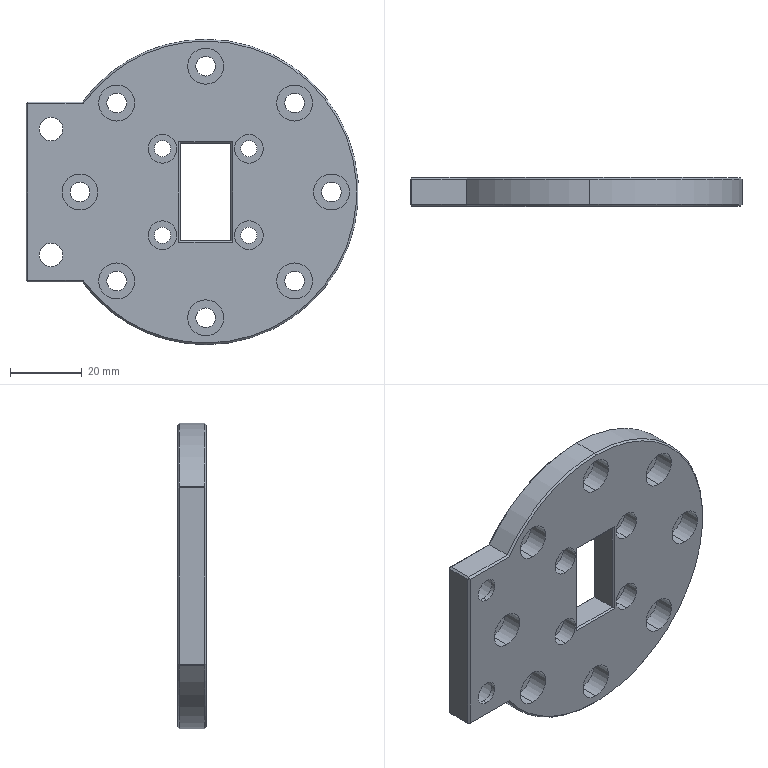Component | SolidWorks | BearingHousingAssembly-1_AirGripperFixingPlate1-1 | 1 solid | 108 faces | box 92.5 x 8 x 85 mm | volume 39781 mm3 | cylinder 59 | plane 43 | cone 6 | commonest cylinder face diameters 10 x16 5.5 x16 8 x8 4.5 x8 11 x4 6.6 x4 85 x3 | material Plain Carbon Steel
build123d program:
from build123d import *

# Parameters (mm, degrees)
SKETCH1_R                                          = 42.5
SKETCH1_W                                          = 27
SKETCH1_H                                          = 14
BOSS_EXTRUDE1_DEPTH                                = 8
HOLE_SIZE_ACCORDING_TO_TYPE_OF_HEXAGON_D           = 5.5
HOLE_SIZE_ACCORDING_TO_TYPE_OF_HEXAGON_CBORE_D     = 10
HOLE_SIZE_ACCORDING_TO_TYPE_OF_HEXAGON_CBORE_DEPTH = 5.7
CIRPATTERN1_COUNT                                  = 8
BOSS_EXTRUDE2_START                                = -8
BOSS_EXTRUDE2_DEPTH                                = 8
HOLE_SIZE_ACCORDING_TO_TYPE_OF_HEX_2_D             = 6.6
HOLE_SIZE_ACCORDING_TO_TYPE_OF_HEX_2_CBORE_D       = 11
HOLE_SIZE_ACCORDING_TO_TYPE_OF_HEX_2_CBORE_DEPTH   = 6.8
CHAMFER1_SIZE                                      = 0.5
CIRPATTERN2_COUNT                                  = 4


with BuildPart() as part:
    # Sketch1 → Boss-Extrude1 (new body)
    with BuildSketch(Plane.XY):
        Circle(SKETCH1_R)
        Rectangle(SKETCH1_W, SKETCH1_H, mode=Mode.SUBTRACT)
    extrude(amount=BOSS_EXTRUDE1_DEPTH)

    # Hole Size _according to_ type of Hexagon (through all)
    with Locations(Plane.XY.offset(8)):
        with Locations((0, 35)):
            hole_size_according_to_type_of_hexagon = CounterBoreHole(HOLE_SIZE_ACCORDING_TO_TYPE_OF_HEXAGON_D / 2, HOLE_SIZE_ACCORDING_TO_TYPE_OF_HEXAGON_CBORE_D / 2, HOLE_SIZE_ACCORDING_TO_TYPE_OF_HEXAGON_CBORE_DEPTH)

    # CirPattern1: Hole Size _according to_ type of Hexagon ×8 about axis
    cirpattern1_axis = Axis((0, 0, 0), (0, 0, 1))
    for i in range(1, CIRPATTERN1_COUNT):
        add(hole_size_according_to_type_of_hexagon.rotate(cirpattern1_axis, i * 360 / CIRPATTERN1_COUNT), mode=Mode.SUBTRACT)

    # Sketch4 → Boss-Extrude2 (add)
    with BuildSketch(Plane.XY.offset(8).offset(BOSS_EXTRUDE2_START)):
        with BuildLine():
            Line((-25, -34.369), (-25, -50))
            Line((-25, -50), (25, -50))
            Line((25, -50), (25, -34.369))
            ThreePointArc((25, -34.369), (0, -42.5), (-25, -34.369))
        make_face()
    extrude(amount=BOSS_EXTRUDE2_DEPTH)

    # Hole Size _according to_ type of Hex 2 (through all)
    with Locations(Plane(origin=(0, 0, 0), x_dir=(-1, 0, 0), z_dir=(0, 0, -1))):
        with Locations((17.5, -43), (-17.5, -43)):
            CounterBoreHole(HOLE_SIZE_ACCORDING_TO_TYPE_OF_HEX_2_D / 2, HOLE_SIZE_ACCORDING_TO_TYPE_OF_HEX_2_CBORE_D / 2, HOLE_SIZE_ACCORDING_TO_TYPE_OF_HEX_2_CBORE_DEPTH)

    # Chamfer1
    chamfer1_edges = [part.edges().sort_by_distance(p)[0] for p in [
        (0, 7, 8),
        (-13.5, 0, 0),
        (0, -7, 0),
        (0, 42.5, 8),
        (0, 42.5, 0),
        (0, -50, 0),
        (25, -50, 4),
        (-25, -42.185, 0),
        (13.5, 0, 0),
        (-25, -50, 4),
        (25, -42.185, 0),
        (0, -50, 8),
        (25, -42.185, 8),
        (-25, -42.185, 8),
        (0, 7, 0),
        (-13.5, 0, 8),
        (0, -7, 8),
        (13.5, 0, 8),
    ]]
    chamfer(chamfer1_edges, length=CHAMFER1_SIZE)

    # Sketch7 → Hole Size_ according to_Type of Hexa 2 (revolve, cut)
    with BuildSketch(Plane(origin=(12.021, 12.021, 8), x_dir=(0, -1, 0), z_dir=(1, 0, 0))):
        Polygon((0, 0), (0, 51.352), (2.25, 50), (2.25, 4.6), (4, 4.6), (4, 0), align=None)
    hole_size_according_to_type_of_hexa_2 = revolve(axis=Axis((12.021, 12.021, 14.35), (0, 0, -1)), mode=Mode.SUBTRACT)

    # CirPattern2: Hole Size_ according to_Type of Hexa 2 ×4 about axis
    cirpattern2_axis = Axis((0, 0, 0), (0, 0, 1))
    for i in range(1, CIRPATTERN2_COUNT):
        add(hole_size_according_to_type_of_hexa_2.rotate(cirpattern2_axis, i * 360 / CIRPATTERN2_COUNT), mode=Mode.SUBTRACT)


solid = part.part

# Placed as in the assembly
solid = solid.moved(Location((-38.666, 129.264, -6), (90, 0, -90)))